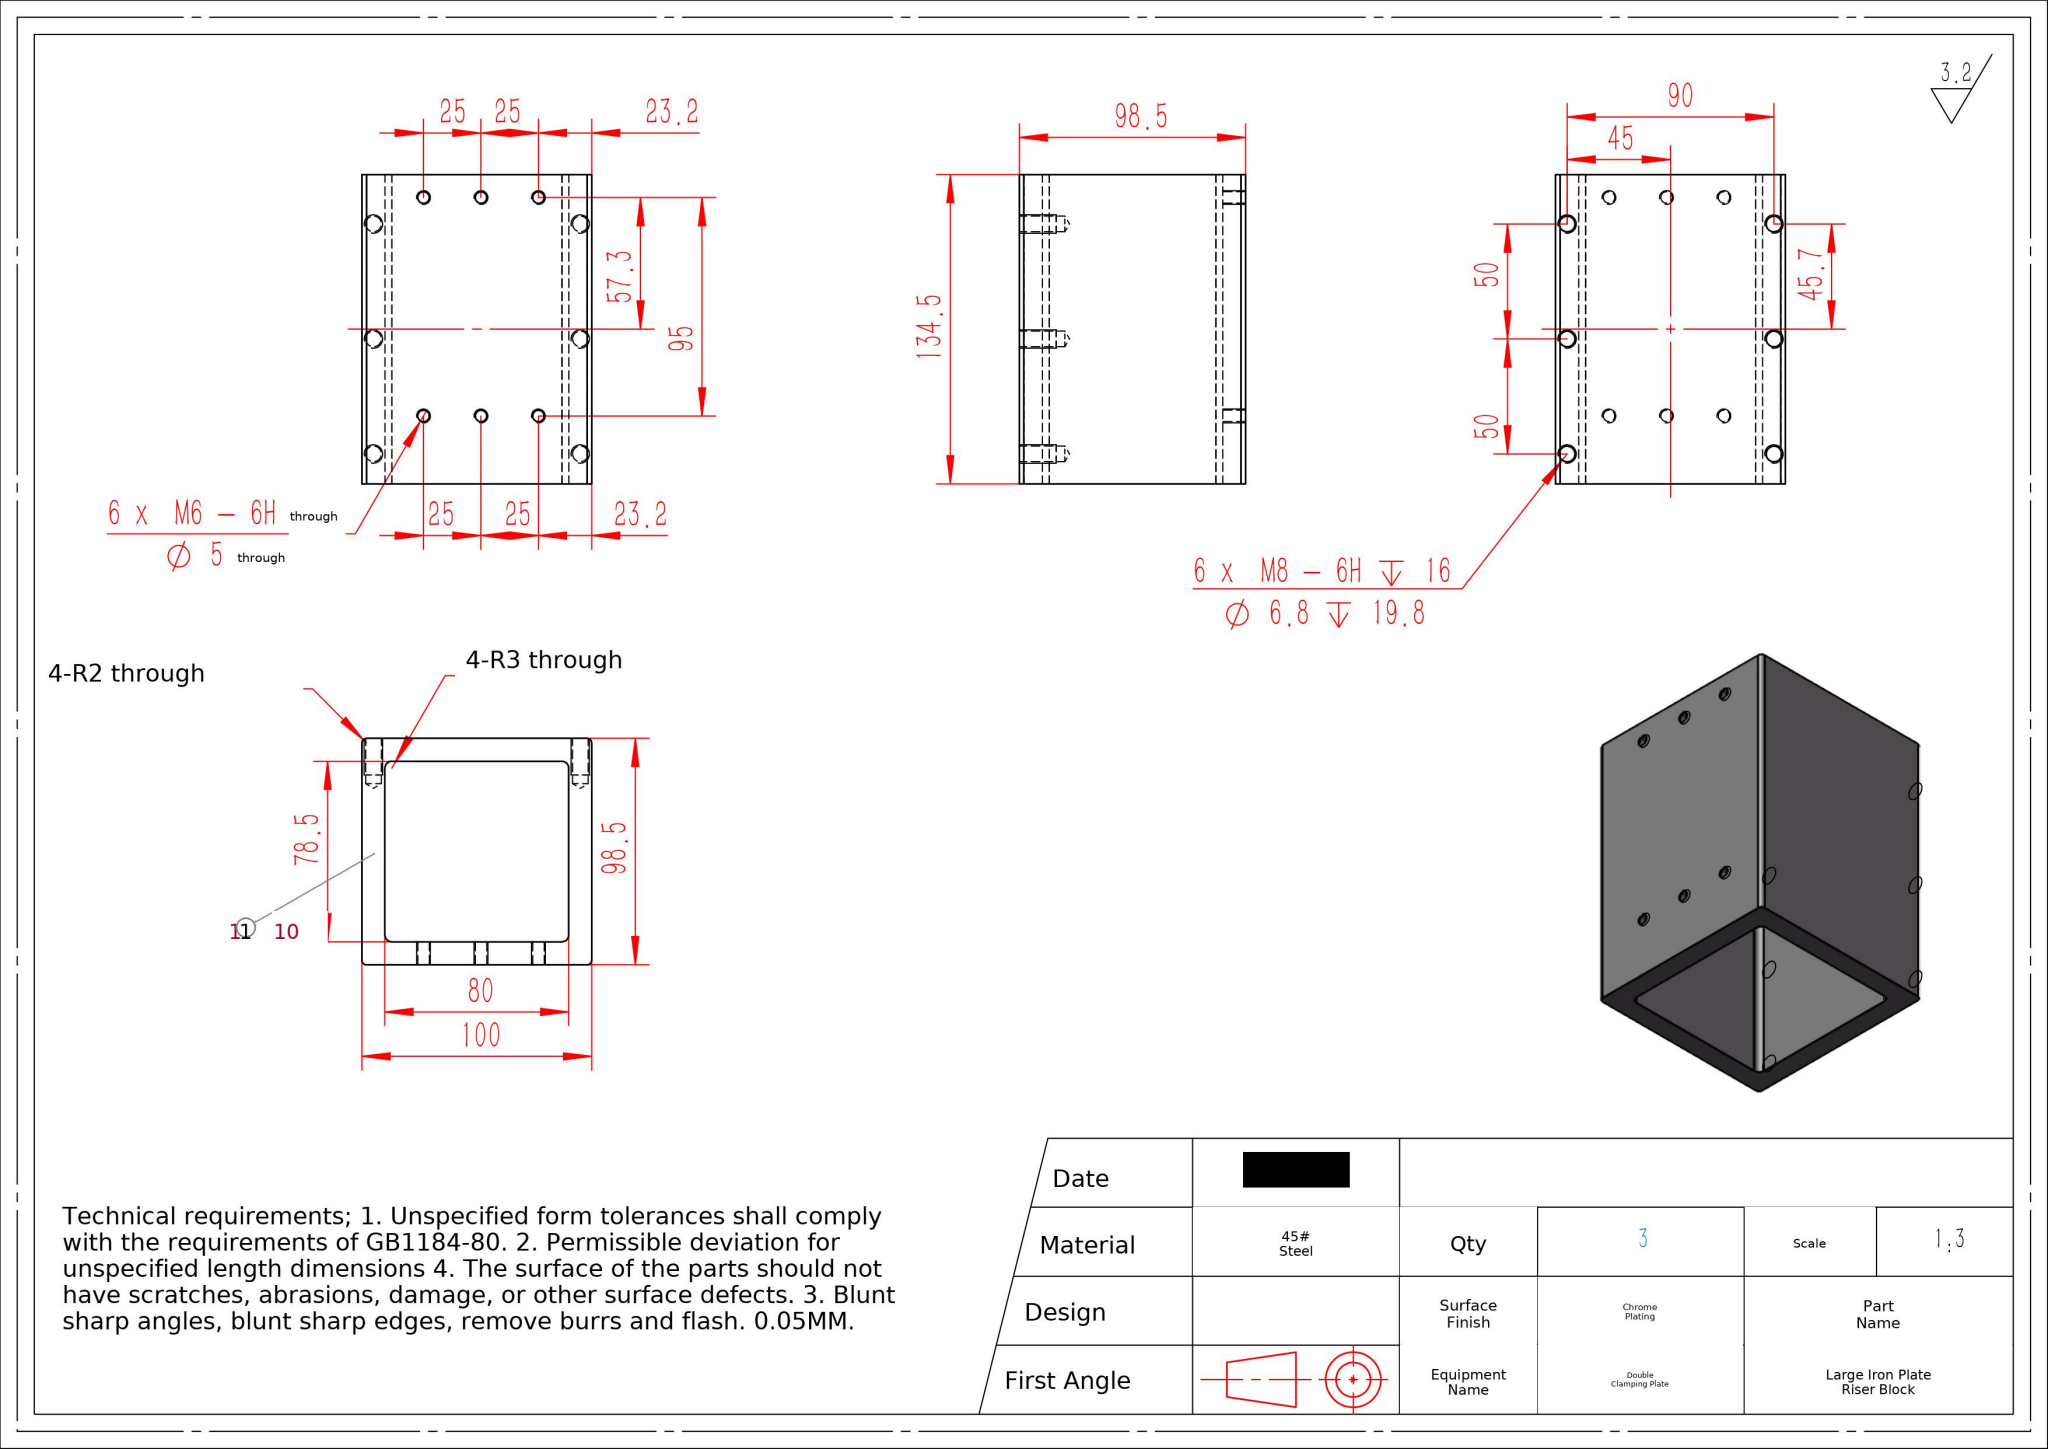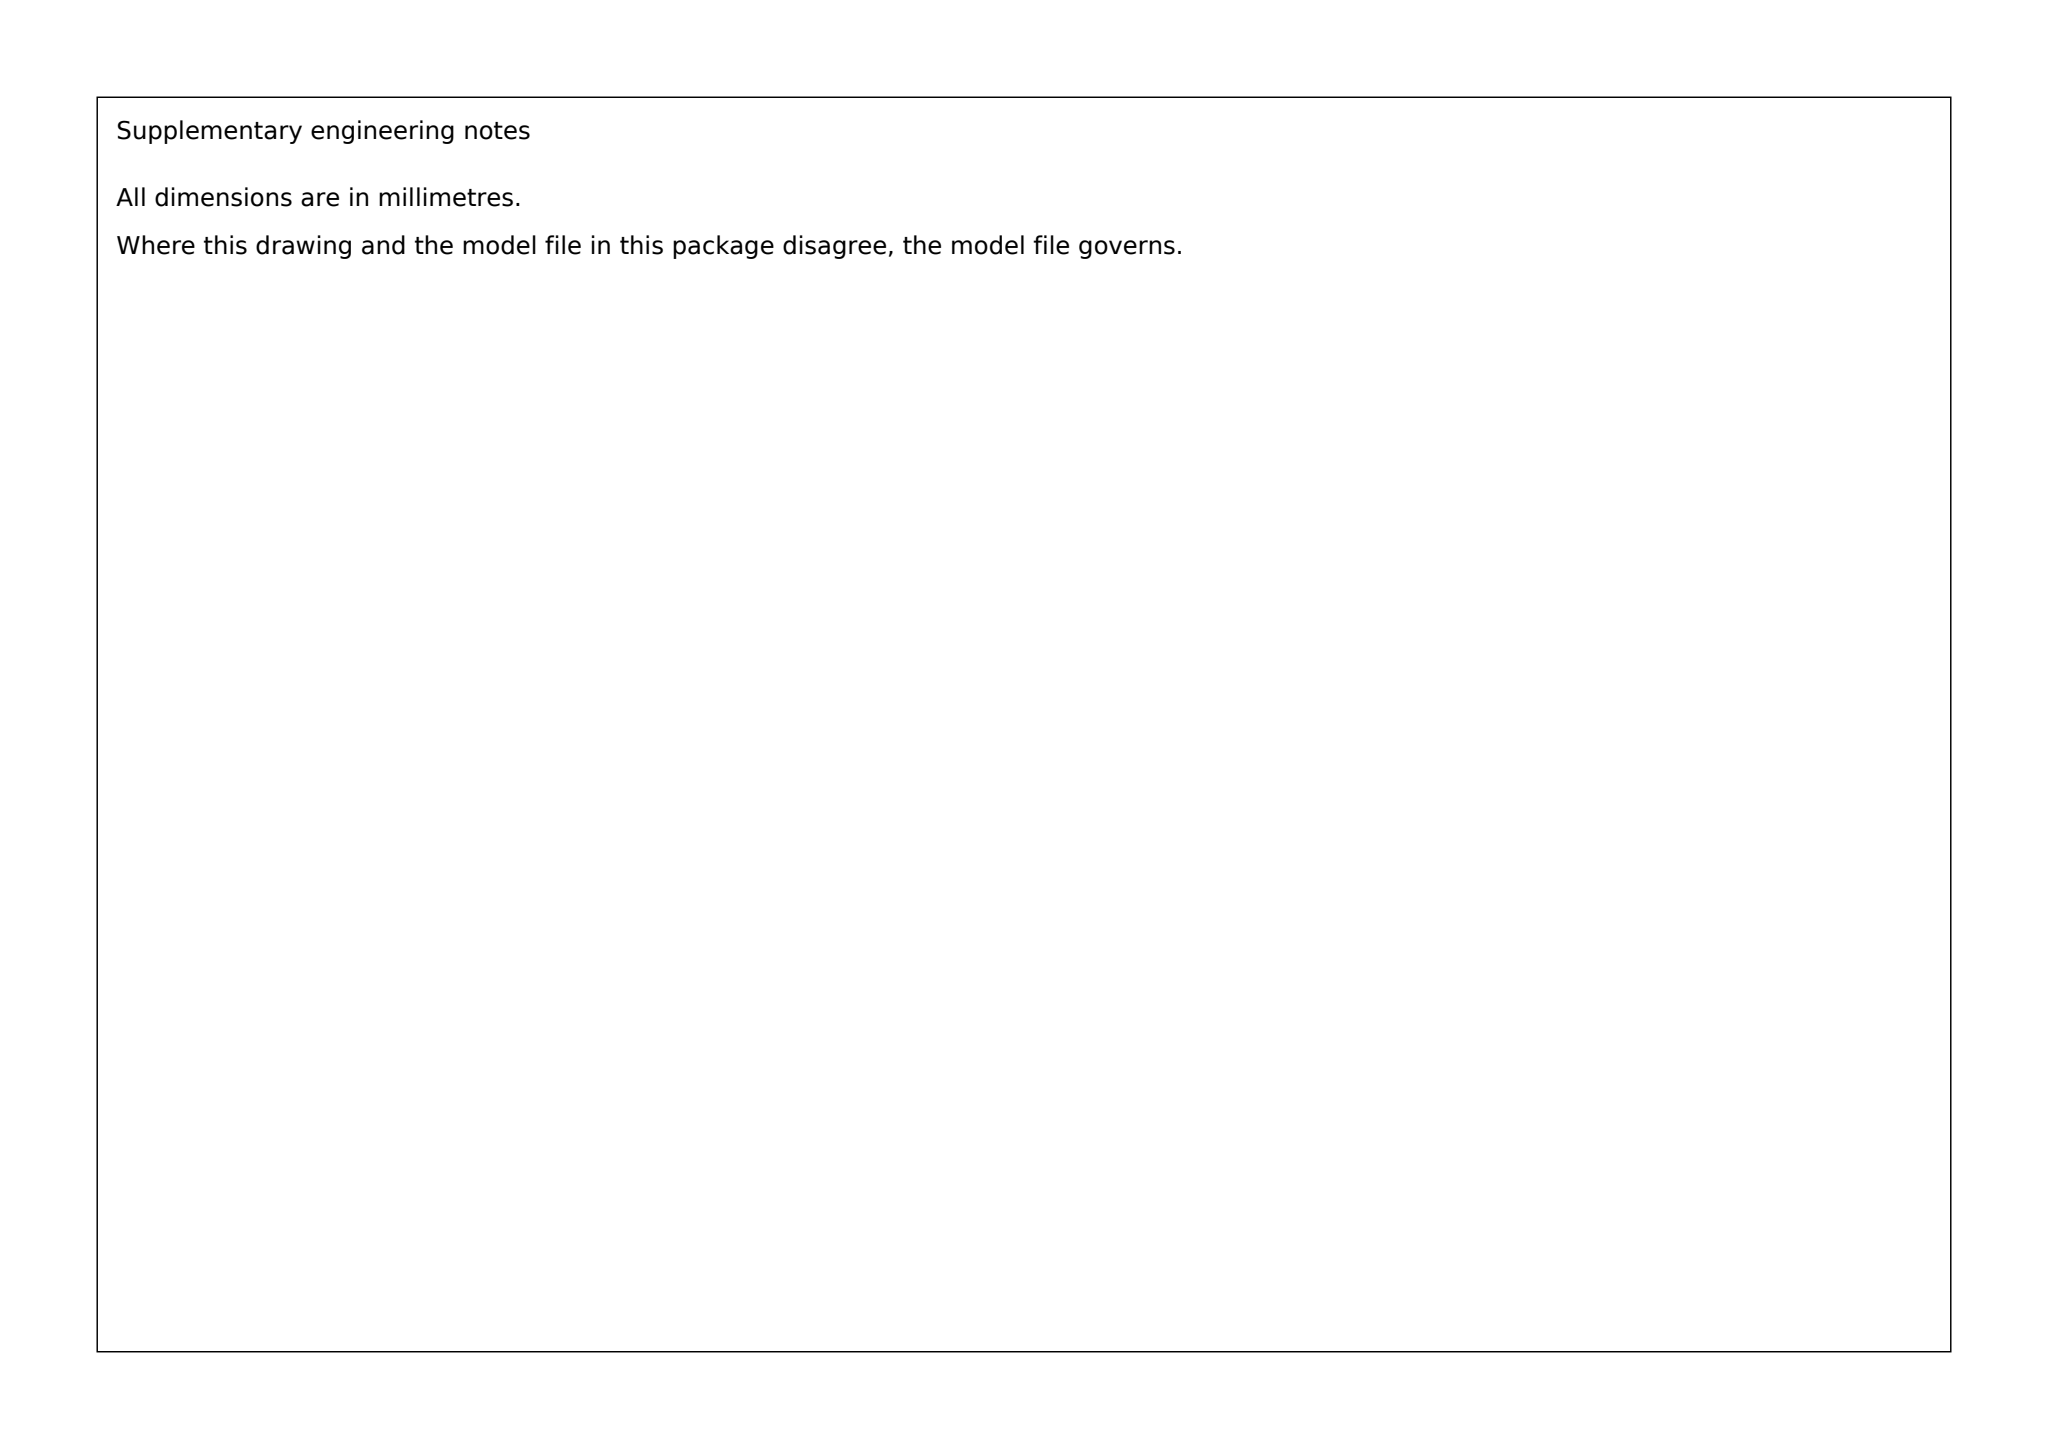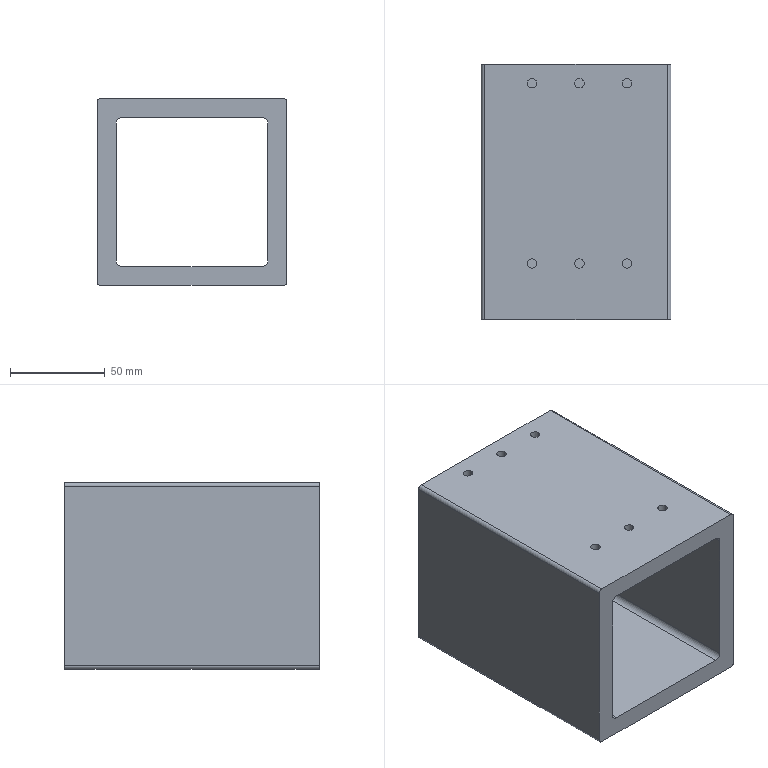Part | SolidWorks | mm | material 45# Steel | 1 solid | 54 faces | box 100 x 134.52 x 98.5 mm | volume 475090 mm3 | cylinder 32 | cone 12 | plane 10 | commonest cylinder face diameters 6.8 x12 5 x12 4 x4 6 x4